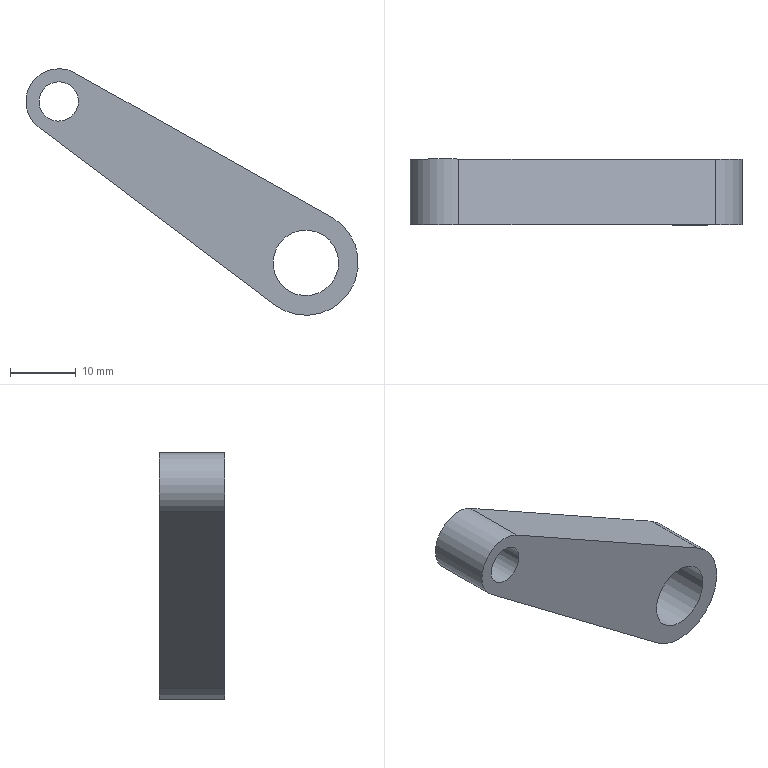Component | NX | JJZ-003_2 | 1 solid | 8 faces | box 50.67 x 10 x 37.61 mm | volume 6193 mm3 | cylinder 4 | plane 4 | commonest cylinder face diameters 10 x2 16 x1 6 x1
STEP:
#1=CARTESIAN_POINT('',(0.,0.,0.));
#2=DIRECTION('',(0.,0.,1.));
#3=DIRECTION('',(1.,0.,0.));
#4=AXIS2_PLACEMENT_3D('',#1,#2,#3);
#5=CARTESIAN_POINT('',(11.419,7.,86.974));
#6=VERTEX_POINT('',#5);
#7=CARTESIAN_POINT('',(2.688,7.,73.609));
#8=VERTEX_POINT('',#7);
#9=CARTESIAN_POINT('',(7.5,7.,80.));
#10=DIRECTION('',(0.,1.,0.));
#11=DIRECTION('',(-0.7797,0.,0.6262));
#12=AXIS2_PLACEMENT_3D('',#9,#10,#11);
#13=CIRCLE('',#12,8.);
#14=CARTESIAN_POINT('',(7.5,17.,80.));
#15=DIRECTION('',(0.,-1.,0.));
#16=DIRECTION('',(0.7797,0.,-0.6262));
#17=AXIS2_PLACEMENT_3D('',#14,#15,#16);
#18=CYLINDRICAL_SURFACE('',#17,8.);
#19=CARTESIAN_POINT('',(3.142,10.));
#20=DIRECTION('',(-1.,0.));
#21=VECTOR('',#20,1.);
#22=LINE('',#19,#21);
#23=(GEOMETRIC_REPRESENTATION_CONTEXT(2)PARAMETRIC_REPRESENTATION_CONTEXT()REPRESENTATION_CONTEXT('',''));
#24=DEFINITIONAL_REPRESENTATION('',(#22),#23);
#25=PCURVE('',#18,#24);
#26=CARTESIAN_POINT('',(7.5,7.,80.));
#27=DIRECTION('',(0.,1.,0.));
#28=DIRECTION('',(-0.7797,0.,0.6262));
#29=AXIS2_PLACEMENT_3D('',#26,#27,#28);
#30=PLANE('',#29);
#31=CARTESIAN_POINT('',(0.,0.));
#32=DIRECTION('',(1.,-0.));
#33=AXIS2_PLACEMENT_2D('',#31,#32);
#34=CIRCLE('',#33,8.);
#35=(GEOMETRIC_REPRESENTATION_CONTEXT(2)PARAMETRIC_REPRESENTATION_CONTEXT()REPRESENTATION_CONTEXT('',''));
#36=DEFINITIONAL_REPRESENTATION('',(#34),#35);
#37=PCURVE('',#30,#36);
#38=SURFACE_CURVE('',#13,(#25,#37),.PCURVE_S1.);
#39=EDGE_CURVE('',#6,#8,#38,.T.);
#40=ORIENTED_EDGE('',*,*,#39,.T.);
#41=CARTESIAN_POINT('',(2.688,17.,73.609));
#42=VERTEX_POINT('',#41);
#43=CARTESIAN_POINT('',(2.688,17.,73.609));
#44=DIRECTION('',(0.,-1.,0.));
#45=VECTOR('',#44,1.);
#46=LINE('',#43,#45);
#47=CARTESIAN_POINT('',(-1.54,0.));
#48=DIRECTION('',(0.,1.));
#49=VECTOR('',#48,1.);
#50=LINE('',#47,#49);
#51=(GEOMETRIC_REPRESENTATION_CONTEXT(2)PARAMETRIC_REPRESENTATION_CONTEXT()REPRESENTATION_CONTEXT('',''));
#52=DEFINITIONAL_REPRESENTATION('',(#50),#51);
#53=PCURVE('',#18,#52);
#54=CARTESIAN_POINT('',(2.688,17.,73.609));
#55=DIRECTION('',(0.6015,0.,0.7988));
#56=DIRECTION('',(0.7988,0.,-0.6015));
#57=AXIS2_PLACEMENT_3D('',#54,#55,#56);
#58=PLANE('',#57);
#59=CARTESIAN_POINT('',(0.,0.));
#60=DIRECTION('',(0.,-1.));
#61=VECTOR('',#60,1.);
#62=LINE('',#59,#61);
#63=(GEOMETRIC_REPRESENTATION_CONTEXT(2)PARAMETRIC_REPRESENTATION_CONTEXT()REPRESENTATION_CONTEXT('',''));
#64=DEFINITIONAL_REPRESENTATION('',(#62),#63);
#65=PCURVE('',#58,#64);
#66=SURFACE_CURVE('',#46,(#53,#65),.PCURVE_S1.);
#67=EDGE_CURVE('',#42,#8,#66,.T.);
#68=ORIENTED_EDGE('',*,*,#67,.F.);
#69=CARTESIAN_POINT('',(11.419,17.,86.974));
#70=VERTEX_POINT('',#69);
#71=CARTESIAN_POINT('',(7.5,17.,80.));
#72=DIRECTION('',(0.,1.,0.));
#73=DIRECTION('',(-0.7797,0.,0.6262));
#74=AXIS2_PLACEMENT_3D('',#71,#72,#73);
#75=CIRCLE('',#74,8.);
#76=CARTESIAN_POINT('',(3.142,0.));
#77=DIRECTION('',(-1.,0.));
#78=VECTOR('',#77,1.);
#79=LINE('',#76,#78);
#80=(GEOMETRIC_REPRESENTATION_CONTEXT(2)PARAMETRIC_REPRESENTATION_CONTEXT()REPRESENTATION_CONTEXT('',''));
#81=DEFINITIONAL_REPRESENTATION('',(#79),#80);
#82=PCURVE('',#18,#81);
#83=CARTESIAN_POINT('',(7.5,17.,80.));
#84=DIRECTION('',(0.,1.,0.));
#85=DIRECTION('',(-0.7797,0.,0.6262));
#86=AXIS2_PLACEMENT_3D('',#83,#84,#85);
#87=PLANE('',#86);
#88=CARTESIAN_POINT('',(0.,0.));
#89=DIRECTION('',(1.,-0.));
#90=AXIS2_PLACEMENT_2D('',#88,#89);
#91=CIRCLE('',#90,8.);
#92=(GEOMETRIC_REPRESENTATION_CONTEXT(2)PARAMETRIC_REPRESENTATION_CONTEXT()REPRESENTATION_CONTEXT('',''));
#93=DEFINITIONAL_REPRESENTATION('',(#91),#92);
#94=PCURVE('',#87,#93);
#95=SURFACE_CURVE('',#75,(#82,#94),.PCURVE_S1.);
#96=EDGE_CURVE('',#70,#42,#95,.T.);
#97=ORIENTED_EDGE('',*,*,#96,.F.);
#98=CARTESIAN_POINT('',(11.419,17.,86.974));
#99=DIRECTION('',(0.,-1.,0.));
#100=VECTOR('',#99,1.);
#101=LINE('',#98,#100);
#102=CARTESIAN_POINT('',(1.735,0.));
#103=DIRECTION('',(0.,1.));
#104=VECTOR('',#103,1.);
#105=LINE('',#102,#104);
#106=(GEOMETRIC_REPRESENTATION_CONTEXT(2)PARAMETRIC_REPRESENTATION_CONTEXT()REPRESENTATION_CONTEXT('',''));
#107=DEFINITIONAL_REPRESENTATION('',(#105),#106);
#108=PCURVE('',#18,#107);
#109=CARTESIAN_POINT('',(-27.723,17.,108.971));
#110=DIRECTION('',(-0.4899,0.,-0.8718));
#111=DIRECTION('',(-0.8718,0.,0.4899));
#112=AXIS2_PLACEMENT_3D('',#109,#110,#111);
#113=PLANE('',#112);
#114=CARTESIAN_POINT('',(-44.9,0.));
#115=DIRECTION('',(0.,-1.));
#116=VECTOR('',#115,1.);
#117=LINE('',#114,#116);
#118=(GEOMETRIC_REPRESENTATION_CONTEXT(2)PARAMETRIC_REPRESENTATION_CONTEXT()REPRESENTATION_CONTEXT('',''));
#119=DEFINITIONAL_REPRESENTATION('',(#117),#118);
#120=PCURVE('',#113,#119);
#121=SURFACE_CURVE('',#101,(#108,#120),.PCURVE_S1.);
#122=EDGE_CURVE('',#70,#6,#121,.T.);
#123=ORIENTED_EDGE('',*,*,#122,.T.);
#124=EDGE_LOOP('',(#40,#68,#97,#123));
#125=FACE_BOUND('',#124,.T.);
#126=ADVANCED_FACE('',(#125),#18,.T.);
#127=CARTESIAN_POINT('',(-33.18,7.,100.618));
#128=VERTEX_POINT('',#127);
#129=CARTESIAN_POINT('',(2.688,7.,73.609));
#130=DIRECTION('',(-0.7988,0.,0.6015));
#131=VECTOR('',#130,1.);
#132=LINE('',#129,#131);
#133=CARTESIAN_POINT('',(0.,-10.));
#134=DIRECTION('',(-1.,0.));
#135=VECTOR('',#134,1.);
#136=LINE('',#133,#135);
#137=(GEOMETRIC_REPRESENTATION_CONTEXT(2)PARAMETRIC_REPRESENTATION_CONTEXT()REPRESENTATION_CONTEXT('',''));
#138=DEFINITIONAL_REPRESENTATION('',(#136),#137);
#139=PCURVE('',#58,#138);
#140=CARTESIAN_POINT('',(-0.2499,-7.996));
#141=DIRECTION('',(0.9995,-0.03124));
#142=VECTOR('',#141,1.);
#143=LINE('',#140,#142);
#144=(GEOMETRIC_REPRESENTATION_CONTEXT(2)PARAMETRIC_REPRESENTATION_CONTEXT()REPRESENTATION_CONTEXT('',''));
#145=DEFINITIONAL_REPRESENTATION('',(#143),#144);
#146=PCURVE('',#30,#145);
#147=SURFACE_CURVE('',#132,(#139,#146),.PCURVE_S1.);
#148=EDGE_CURVE('',#8,#128,#147,.T.);
#149=ORIENTED_EDGE('',*,*,#148,.T.);
#150=CARTESIAN_POINT('',(-33.18,17.,100.618));
#151=VERTEX_POINT('',#150);
#152=CARTESIAN_POINT('',(-33.18,17.,100.618));
#153=DIRECTION('',(0.,-1.,0.));
#154=VECTOR('',#153,1.);
#155=LINE('',#152,#154);
#156=CARTESIAN_POINT('',(-44.9,0.));
#157=DIRECTION('',(0.,-1.));
#158=VECTOR('',#157,1.);
#159=LINE('',#156,#158);
#160=(GEOMETRIC_REPRESENTATION_CONTEXT(2)PARAMETRIC_REPRESENTATION_CONTEXT()REPRESENTATION_CONTEXT('',''));
#161=DEFINITIONAL_REPRESENTATION('',(#159),#160);
#162=PCURVE('',#58,#161);
#163=CARTESIAN_POINT('',(-30.173,17.,104.612));
#164=DIRECTION('',(0.,-1.,0.));
#165=DIRECTION('',(0.7797,0.,-0.6262));
#166=AXIS2_PLACEMENT_3D('',#163,#164,#165);
#167=CYLINDRICAL_SURFACE('',#166,5.);
#168=CARTESIAN_POINT('',(4.744,0.));
#169=DIRECTION('',(0.,1.));
#170=VECTOR('',#169,1.);
#171=LINE('',#168,#170);
#172=(GEOMETRIC_REPRESENTATION_CONTEXT(2)PARAMETRIC_REPRESENTATION_CONTEXT()REPRESENTATION_CONTEXT('',''));
#173=DEFINITIONAL_REPRESENTATION('',(#171),#172);
#174=PCURVE('',#167,#173);
#175=SURFACE_CURVE('',#155,(#162,#174),.PCURVE_S1.);
#176=EDGE_CURVE('',#151,#128,#175,.T.);
#177=ORIENTED_EDGE('',*,*,#176,.F.);
#178=CARTESIAN_POINT('',(2.688,17.,73.609));
#179=DIRECTION('',(-0.7988,0.,0.6015));
#180=VECTOR('',#179,1.);
#181=LINE('',#178,#180);
#182=CARTESIAN_POINT('',(0.,0.));
#183=DIRECTION('',(-1.,0.));
#184=VECTOR('',#183,1.);
#185=LINE('',#182,#184);
#186=(GEOMETRIC_REPRESENTATION_CONTEXT(2)PARAMETRIC_REPRESENTATION_CONTEXT()REPRESENTATION_CONTEXT('',''));
#187=DEFINITIONAL_REPRESENTATION('',(#185),#186);
#188=PCURVE('',#58,#187);
#189=CARTESIAN_POINT('',(-0.2499,-7.996));
#190=DIRECTION('',(0.9995,-0.03124));
#191=VECTOR('',#190,1.);
#192=LINE('',#189,#191);
#193=(GEOMETRIC_REPRESENTATION_CONTEXT(2)PARAMETRIC_REPRESENTATION_CONTEXT()REPRESENTATION_CONTEXT('',''));
#194=DEFINITIONAL_REPRESENTATION('',(#192),#193);
#195=PCURVE('',#87,#194);
#196=SURFACE_CURVE('',#181,(#188,#195),.PCURVE_S1.);
#197=EDGE_CURVE('',#42,#151,#196,.T.);
#198=ORIENTED_EDGE('',*,*,#197,.F.);
#199=ORIENTED_EDGE('',*,*,#67,.T.);
#200=EDGE_LOOP('',(#149,#177,#198,#199));
#201=FACE_BOUND('',#200,.T.);
#202=ADVANCED_FACE('',(#201),#58,.F.);
#203=CARTESIAN_POINT('',(-27.723,7.,108.971));
#204=VERTEX_POINT('',#203);
#205=CARTESIAN_POINT('',(-30.173,7.,104.612));
#206=DIRECTION('',(0.,1.,0.));
#207=DIRECTION('',(-0.7797,0.,0.6262));
#208=AXIS2_PLACEMENT_3D('',#205,#206,#207);
#209=CIRCLE('',#208,5.);
#210=CARTESIAN_POINT('',(9.425,10.));
#211=DIRECTION('',(-1.,0.));
#212=VECTOR('',#211,1.);
#213=LINE('',#210,#212);
#214=(GEOMETRIC_REPRESENTATION_CONTEXT(2)PARAMETRIC_REPRESENTATION_CONTEXT()REPRESENTATION_CONTEXT('',''));
#215=DEFINITIONAL_REPRESENTATION('',(#213),#214);
#216=PCURVE('',#167,#215);
#217=CARTESIAN_POINT('',(44.784,-4.401));
#218=DIRECTION('',(1.,-0.));
#219=AXIS2_PLACEMENT_2D('',#217,#218);
#220=CIRCLE('',#219,5.);
#221=(GEOMETRIC_REPRESENTATION_CONTEXT(2)PARAMETRIC_REPRESENTATION_CONTEXT()REPRESENTATION_CONTEXT('',''));
#222=DEFINITIONAL_REPRESENTATION('',(#220),#221);
#223=PCURVE('',#30,#222);
#224=SURFACE_CURVE('',#209,(#216,#223),.PCURVE_S1.);
#225=EDGE_CURVE('',#128,#204,#224,.T.);
#226=ORIENTED_EDGE('',*,*,#225,.T.);
#227=CARTESIAN_POINT('',(-27.723,17.,108.971));
#228=VERTEX_POINT('',#227);
#229=CARTESIAN_POINT('',(-27.723,17.,108.971));
#230=DIRECTION('',(0.,-1.,0.));
#231=VECTOR('',#230,1.);
#232=LINE('',#229,#231);
#233=CARTESIAN_POINT('',(1.735,0.));
#234=DIRECTION('',(0.,1.));
#235=VECTOR('',#234,1.);
#236=LINE('',#233,#235);
#237=(GEOMETRIC_REPRESENTATION_CONTEXT(2)PARAMETRIC_REPRESENTATION_CONTEXT()REPRESENTATION_CONTEXT('',''));
#238=DEFINITIONAL_REPRESENTATION('',(#236),#237);
#239=PCURVE('',#167,#238);
#240=CARTESIAN_POINT('',(0.,0.));
#241=DIRECTION('',(0.,-1.));
#242=VECTOR('',#241,1.);
#243=LINE('',#240,#242);
#244=(GEOMETRIC_REPRESENTATION_CONTEXT(2)PARAMETRIC_REPRESENTATION_CONTEXT()REPRESENTATION_CONTEXT('',''));
#245=DEFINITIONAL_REPRESENTATION('',(#243),#244);
#246=PCURVE('',#113,#245);
#247=SURFACE_CURVE('',#232,(#239,#246),.PCURVE_S1.);
#248=EDGE_CURVE('',#228,#204,#247,.T.);
#249=ORIENTED_EDGE('',*,*,#248,.F.);
#250=CARTESIAN_POINT('',(-30.173,17.,104.612));
#251=DIRECTION('',(0.,1.,0.));
#252=DIRECTION('',(-0.7797,0.,0.6262));
#253=AXIS2_PLACEMENT_3D('',#250,#251,#252);
#254=CIRCLE('',#253,5.);
#255=CARTESIAN_POINT('',(9.425,0.));
#256=DIRECTION('',(-1.,0.));
#257=VECTOR('',#256,1.);
#258=LINE('',#255,#257);
#259=(GEOMETRIC_REPRESENTATION_CONTEXT(2)PARAMETRIC_REPRESENTATION_CONTEXT()REPRESENTATION_CONTEXT('',''));
#260=DEFINITIONAL_REPRESENTATION('',(#258),#259);
#261=PCURVE('',#167,#260);
#262=CARTESIAN_POINT('',(44.784,-4.401));
#263=DIRECTION('',(1.,-0.));
#264=AXIS2_PLACEMENT_2D('',#262,#263);
#265=CIRCLE('',#264,5.);
#266=(GEOMETRIC_REPRESENTATION_CONTEXT(2)PARAMETRIC_REPRESENTATION_CONTEXT()REPRESENTATION_CONTEXT('',''));
#267=DEFINITIONAL_REPRESENTATION('',(#265),#266);
#268=PCURVE('',#87,#267);
#269=SURFACE_CURVE('',#254,(#261,#268),.PCURVE_S1.);
#270=EDGE_CURVE('',#151,#228,#269,.T.);
#271=ORIENTED_EDGE('',*,*,#270,.F.);
#272=ORIENTED_EDGE('',*,*,#176,.T.);
#273=EDGE_LOOP('',(#226,#249,#271,#272));
#274=FACE_BOUND('',#273,.T.);
#275=ADVANCED_FACE('',(#274),#167,.T.);
#276=CARTESIAN_POINT('',(3.602,17.,83.131));
#277=VERTEX_POINT('',#276);
#278=CARTESIAN_POINT('',(7.5,17.,80.));
#279=DIRECTION('',(0.,1.,0.));
#280=DIRECTION('',(-0.7797,0.,0.6262));
#281=AXIS2_PLACEMENT_3D('',#278,#279,#280);
#282=CIRCLE('',#281,5.);
#283=CARTESIAN_POINT('',(7.5,17.,80.));
#284=DIRECTION('',(0.,-1.,0.));
#285=DIRECTION('',(0.7797,0.,-0.6262));
#286=AXIS2_PLACEMENT_3D('',#283,#284,#285);
#287=CYLINDRICAL_SURFACE('',#286,5.);
#288=CARTESIAN_POINT('',(9.425,0.));
#289=DIRECTION('',(-1.,0.));
#290=VECTOR('',#289,1.);
#291=LINE('',#288,#290);
#292=(GEOMETRIC_REPRESENTATION_CONTEXT(2)PARAMETRIC_REPRESENTATION_CONTEXT()REPRESENTATION_CONTEXT('',''));
#293=DEFINITIONAL_REPRESENTATION('',(#291),#292);
#294=PCURVE('',#287,#293);
#295=CARTESIAN_POINT('',(0.,0.));
#296=DIRECTION('',(1.,-0.));
#297=AXIS2_PLACEMENT_2D('',#295,#296);
#298=CIRCLE('',#297,5.);
#299=(GEOMETRIC_REPRESENTATION_CONTEXT(2)PARAMETRIC_REPRESENTATION_CONTEXT()REPRESENTATION_CONTEXT('',''));
#300=DEFINITIONAL_REPRESENTATION('',(#298),#299);
#301=PCURVE('',#87,#300);
#302=SURFACE_CURVE('',#282,(#294,#301),.PCURVE_S1.);
#303=EDGE_CURVE('',#277,#277,#302,.T.);
#304=ORIENTED_EDGE('',*,*,#303,.F.);
#305=CARTESIAN_POINT('',(3.602,7.,83.131));
#306=VERTEX_POINT('',#305);
#307=CARTESIAN_POINT('',(3.602,17.,83.131));
#308=CARTESIAN_POINT('',(3.602,7.,83.131));
#309=B_SPLINE_CURVE_WITH_KNOTS('',1,(#307,#308),.UNSPECIFIED.,.F.,.F.,(2,2),(0.,10.),.PIECEWISE_BEZIER_KNOTS.);
#310=CARTESIAN_POINT('',(9.425,0.));
#311=DIRECTION('',(0.,1.));
#312=VECTOR('',#311,1.);
#313=LINE('',#310,#312);
#314=(GEOMETRIC_REPRESENTATION_CONTEXT(2)PARAMETRIC_REPRESENTATION_CONTEXT()REPRESENTATION_CONTEXT('',''));
#315=DEFINITIONAL_REPRESENTATION('',(#313),#314);
#316=PCURVE('',#287,#315);
#317=CARTESIAN_POINT('',(3.142,0.));
#318=DIRECTION('',(0.,1.));
#319=VECTOR('',#318,1.);
#320=LINE('',#317,#319);
#321=(GEOMETRIC_REPRESENTATION_CONTEXT(2)PARAMETRIC_REPRESENTATION_CONTEXT()REPRESENTATION_CONTEXT('',''));
#322=DEFINITIONAL_REPRESENTATION('',(#320),#321);
#323=PCURVE('',#287,#322);
#324=SEAM_CURVE('',#309,(#316,#323),.PCURVE_S1.);
#325=EDGE_CURVE('',#277,#306,#324,.T.);
#326=ORIENTED_EDGE('',*,*,#325,.T.);
#327=CARTESIAN_POINT('',(7.5,7.,80.));
#328=DIRECTION('',(0.,1.,0.));
#329=DIRECTION('',(-0.7797,0.,0.6262));
#330=AXIS2_PLACEMENT_3D('',#327,#328,#329);
#331=CIRCLE('',#330,5.);
#332=CARTESIAN_POINT('',(9.425,10.));
#333=DIRECTION('',(-1.,0.));
#334=VECTOR('',#333,1.);
#335=LINE('',#332,#334);
#336=(GEOMETRIC_REPRESENTATION_CONTEXT(2)PARAMETRIC_REPRESENTATION_CONTEXT()REPRESENTATION_CONTEXT('',''));
#337=DEFINITIONAL_REPRESENTATION('',(#335),#336);
#338=PCURVE('',#287,#337);
#339=CARTESIAN_POINT('',(0.,0.));
#340=DIRECTION('',(1.,-0.));
#341=AXIS2_PLACEMENT_2D('',#339,#340);
#342=CIRCLE('',#341,5.);
#343=(GEOMETRIC_REPRESENTATION_CONTEXT(2)PARAMETRIC_REPRESENTATION_CONTEXT()REPRESENTATION_CONTEXT('',''));
#344=DEFINITIONAL_REPRESENTATION('',(#342),#343);
#345=PCURVE('',#30,#344);
#346=SURFACE_CURVE('',#331,(#338,#345),.PCURVE_S1.);
#347=EDGE_CURVE('',#306,#306,#346,.T.);
#348=ORIENTED_EDGE('',*,*,#347,.T.);
#349=ORIENTED_EDGE('',*,*,#325,.F.);
#350=EDGE_LOOP('',(#304,#326,#348,#349));
#351=FACE_BOUND('',#350,.F.);
#352=ADVANCED_FACE('',(#351),#287,.F.);
#353=CARTESIAN_POINT('',(-27.723,7.,108.971));
#354=DIRECTION('',(0.8718,0.,-0.4899));
#355=VECTOR('',#354,1.);
#356=LINE('',#353,#355);
#357=CARTESIAN_POINT('',(0.,-10.));
#358=DIRECTION('',(-1.,0.));
#359=VECTOR('',#358,1.);
#360=LINE('',#357,#359);
#361=(GEOMETRIC_REPRESENTATION_CONTEXT(2)PARAMETRIC_REPRESENTATION_CONTEXT()REPRESENTATION_CONTEXT('',''));
#362=DEFINITIONAL_REPRESENTATION('',(#360),#361);
#363=PCURVE('',#113,#362);
#364=CARTESIAN_POINT('',(45.604,0.531));
#365=DIRECTION('',(-0.9865,0.1639));
#366=VECTOR('',#365,1.);
#367=LINE('',#364,#366);
#368=(GEOMETRIC_REPRESENTATION_CONTEXT(2)PARAMETRIC_REPRESENTATION_CONTEXT()REPRESENTATION_CONTEXT('',''));
#369=DEFINITIONAL_REPRESENTATION('',(#367),#368);
#370=PCURVE('',#30,#369);
#371=SURFACE_CURVE('',#356,(#363,#370),.PCURVE_S1.);
#372=EDGE_CURVE('',#204,#6,#371,.T.);
#373=ORIENTED_EDGE('',*,*,#372,.T.);
#374=ORIENTED_EDGE('',*,*,#122,.F.);
#375=CARTESIAN_POINT('',(-27.723,17.,108.971));
#376=DIRECTION('',(0.8718,0.,-0.4899));
#377=VECTOR('',#376,1.);
#378=LINE('',#375,#377);
#379=CARTESIAN_POINT('',(0.,0.));
#380=DIRECTION('',(-1.,0.));
#381=VECTOR('',#380,1.);
#382=LINE('',#379,#381);
#383=(GEOMETRIC_REPRESENTATION_CONTEXT(2)PARAMETRIC_REPRESENTATION_CONTEXT()REPRESENTATION_CONTEXT('',''));
#384=DEFINITIONAL_REPRESENTATION('',(#382),#383);
#385=PCURVE('',#113,#384);
#386=CARTESIAN_POINT('',(45.604,0.531));
#387=DIRECTION('',(-0.9865,0.1639));
#388=VECTOR('',#387,1.);
#389=LINE('',#386,#388);
#390=(GEOMETRIC_REPRESENTATION_CONTEXT(2)PARAMETRIC_REPRESENTATION_CONTEXT()REPRESENTATION_CONTEXT('',''));
#391=DEFINITIONAL_REPRESENTATION('',(#389),#390);
#392=PCURVE('',#87,#391);
#393=SURFACE_CURVE('',#378,(#385,#392),.PCURVE_S1.);
#394=EDGE_CURVE('',#228,#70,#393,.T.);
#395=ORIENTED_EDGE('',*,*,#394,.F.);
#396=ORIENTED_EDGE('',*,*,#248,.T.);
#397=EDGE_LOOP('',(#373,#374,#395,#396));
#398=FACE_BOUND('',#397,.T.);
#399=ADVANCED_FACE('',(#398),#113,.F.);
#400=CARTESIAN_POINT('',(-32.512,17.,106.491));
#401=VERTEX_POINT('',#400);
#402=CARTESIAN_POINT('',(-30.173,17.,104.612));
#403=DIRECTION('',(0.,1.,0.));
#404=DIRECTION('',(-0.7797,0.,0.6262));
#405=AXIS2_PLACEMENT_3D('',#402,#403,#404);
#406=CIRCLE('',#405,3.);
#407=CARTESIAN_POINT('',(-30.173,17.,104.612));
#408=DIRECTION('',(0.,-1.,0.));
#409=DIRECTION('',(0.7797,0.,-0.6262));
#410=AXIS2_PLACEMENT_3D('',#407,#408,#409);
#411=CYLINDRICAL_SURFACE('',#410,3.);
#412=CARTESIAN_POINT('',(9.425,0.));
#413=DIRECTION('',(-1.,0.));
#414=VECTOR('',#413,1.);
#415=LINE('',#412,#414);
#416=(GEOMETRIC_REPRESENTATION_CONTEXT(2)PARAMETRIC_REPRESENTATION_CONTEXT()REPRESENTATION_CONTEXT('',''));
#417=DEFINITIONAL_REPRESENTATION('',(#415),#416);
#418=PCURVE('',#411,#417);
#419=CARTESIAN_POINT('',(44.784,-4.401));
#420=DIRECTION('',(1.,0.));
#421=AXIS2_PLACEMENT_2D('',#419,#420);
#422=CIRCLE('',#421,3.);
#423=(GEOMETRIC_REPRESENTATION_CONTEXT(2)PARAMETRIC_REPRESENTATION_CONTEXT()REPRESENTATION_CONTEXT('',''));
#424=DEFINITIONAL_REPRESENTATION('',(#422),#423);
#425=PCURVE('',#87,#424);
#426=SURFACE_CURVE('',#406,(#418,#425),.PCURVE_S1.);
#427=EDGE_CURVE('',#401,#401,#426,.T.);
#428=ORIENTED_EDGE('',*,*,#427,.F.);
#429=CARTESIAN_POINT('',(-32.512,7.,106.491));
#430=VERTEX_POINT('',#429);
#431=CARTESIAN_POINT('',(-32.512,17.,106.491));
#432=CARTESIAN_POINT('',(-32.512,7.,106.491));
#433=B_SPLINE_CURVE_WITH_KNOTS('',1,(#431,#432),.UNSPECIFIED.,.F.,.F.,(2,2),(0.,10.),.PIECEWISE_BEZIER_KNOTS.);
#434=CARTESIAN_POINT('',(9.425,0.));
#435=DIRECTION('',(0.,1.));
#436=VECTOR('',#435,1.);
#437=LINE('',#434,#436);
#438=(GEOMETRIC_REPRESENTATION_CONTEXT(2)PARAMETRIC_REPRESENTATION_CONTEXT()REPRESENTATION_CONTEXT('',''));
#439=DEFINITIONAL_REPRESENTATION('',(#437),#438);
#440=PCURVE('',#411,#439);
#441=CARTESIAN_POINT('',(3.142,0.));
#442=DIRECTION('',(0.,1.));
#443=VECTOR('',#442,1.);
#444=LINE('',#441,#443);
#445=(GEOMETRIC_REPRESENTATION_CONTEXT(2)PARAMETRIC_REPRESENTATION_CONTEXT()REPRESENTATION_CONTEXT('',''));
#446=DEFINITIONAL_REPRESENTATION('',(#444),#445);
#447=PCURVE('',#411,#446);
#448=SEAM_CURVE('',#433,(#440,#447),.PCURVE_S1.);
#449=EDGE_CURVE('',#401,#430,#448,.T.);
#450=ORIENTED_EDGE('',*,*,#449,.T.);
#451=CARTESIAN_POINT('',(-30.173,7.,104.612));
#452=DIRECTION('',(0.,1.,0.));
#453=DIRECTION('',(-0.7797,0.,0.6262));
#454=AXIS2_PLACEMENT_3D('',#451,#452,#453);
#455=CIRCLE('',#454,3.);
#456=CARTESIAN_POINT('',(9.425,10.));
#457=DIRECTION('',(-1.,0.));
#458=VECTOR('',#457,1.);
#459=LINE('',#456,#458);
#460=(GEOMETRIC_REPRESENTATION_CONTEXT(2)PARAMETRIC_REPRESENTATION_CONTEXT()REPRESENTATION_CONTEXT('',''));
#461=DEFINITIONAL_REPRESENTATION('',(#459),#460);
#462=PCURVE('',#411,#461);
#463=CARTESIAN_POINT('',(44.784,-4.401));
#464=DIRECTION('',(1.,0.));
#465=AXIS2_PLACEMENT_2D('',#463,#464);
#466=CIRCLE('',#465,3.);
#467=(GEOMETRIC_REPRESENTATION_CONTEXT(2)PARAMETRIC_REPRESENTATION_CONTEXT()REPRESENTATION_CONTEXT('',''));
#468=DEFINITIONAL_REPRESENTATION('',(#466),#467);
#469=PCURVE('',#30,#468);
#470=SURFACE_CURVE('',#455,(#462,#469),.PCURVE_S1.);
#471=EDGE_CURVE('',#430,#430,#470,.T.);
#472=ORIENTED_EDGE('',*,*,#471,.T.);
#473=ORIENTED_EDGE('',*,*,#449,.F.);
#474=EDGE_LOOP('',(#428,#450,#472,#473));
#475=FACE_BOUND('',#474,.F.);
#476=ADVANCED_FACE('',(#475),#411,.F.);
#477=ORIENTED_EDGE('',*,*,#96,.T.);
#478=ORIENTED_EDGE('',*,*,#197,.T.);
#479=ORIENTED_EDGE('',*,*,#270,.T.);
#480=ORIENTED_EDGE('',*,*,#394,.T.);
#481=EDGE_LOOP('',(#477,#478,#479,#480));
#482=FACE_BOUND('',#481,.T.);
#483=ORIENTED_EDGE('',*,*,#303,.F.);
#484=EDGE_LOOP('',(#483));
#485=FACE_BOUND('',#484,.T.);
#486=ORIENTED_EDGE('',*,*,#427,.F.);
#487=EDGE_LOOP('',(#486));
#488=FACE_BOUND('',#487,.T.);
#489=ADVANCED_FACE('',(#482,#485,#488),#87,.T.);
#490=ORIENTED_EDGE('',*,*,#39,.F.);
#491=ORIENTED_EDGE('',*,*,#372,.F.);
#492=ORIENTED_EDGE('',*,*,#225,.F.);
#493=ORIENTED_EDGE('',*,*,#148,.F.);
#494=EDGE_LOOP('',(#490,#491,#492,#493));
#495=FACE_BOUND('',#494,.T.);
#496=ORIENTED_EDGE('',*,*,#347,.T.);
#497=EDGE_LOOP('',(#496));
#498=FACE_BOUND('',#497,.T.);
#499=ORIENTED_EDGE('',*,*,#471,.T.);
#500=EDGE_LOOP('',(#499));
#501=FACE_BOUND('',#500,.T.);
#502=ADVANCED_FACE('',(#495,#498,#501),#30,.F.);
#503=CLOSED_SHELL('',(#126,#202,#275,#352,#399,#476,#489,#502));
#504=MANIFOLD_SOLID_BREP('',#503);
#505=(LENGTH_UNIT()NAMED_UNIT(*)SI_UNIT(.MILLI.,.METRE.));
#506=UNCERTAINTY_MEASURE_WITH_UNIT(LENGTH_MEASURE(0.000002),#505,'','');
#507=(NAMED_UNIT(*)PLANE_ANGLE_UNIT()SI_UNIT($,.RADIAN.));
#508=(NAMED_UNIT(*)SI_UNIT($,.STERADIAN.)SOLID_ANGLE_UNIT());
#509=(GEOMETRIC_REPRESENTATION_CONTEXT(3)GLOBAL_UNCERTAINTY_ASSIGNED_CONTEXT((#506))GLOBAL_UNIT_ASSIGNED_CONTEXT((#505,#507,#508))REPRESENTATION_CONTEXT('',''));
#510=ADVANCED_BREP_SHAPE_REPRESENTATION('',(#4,#504),#509);